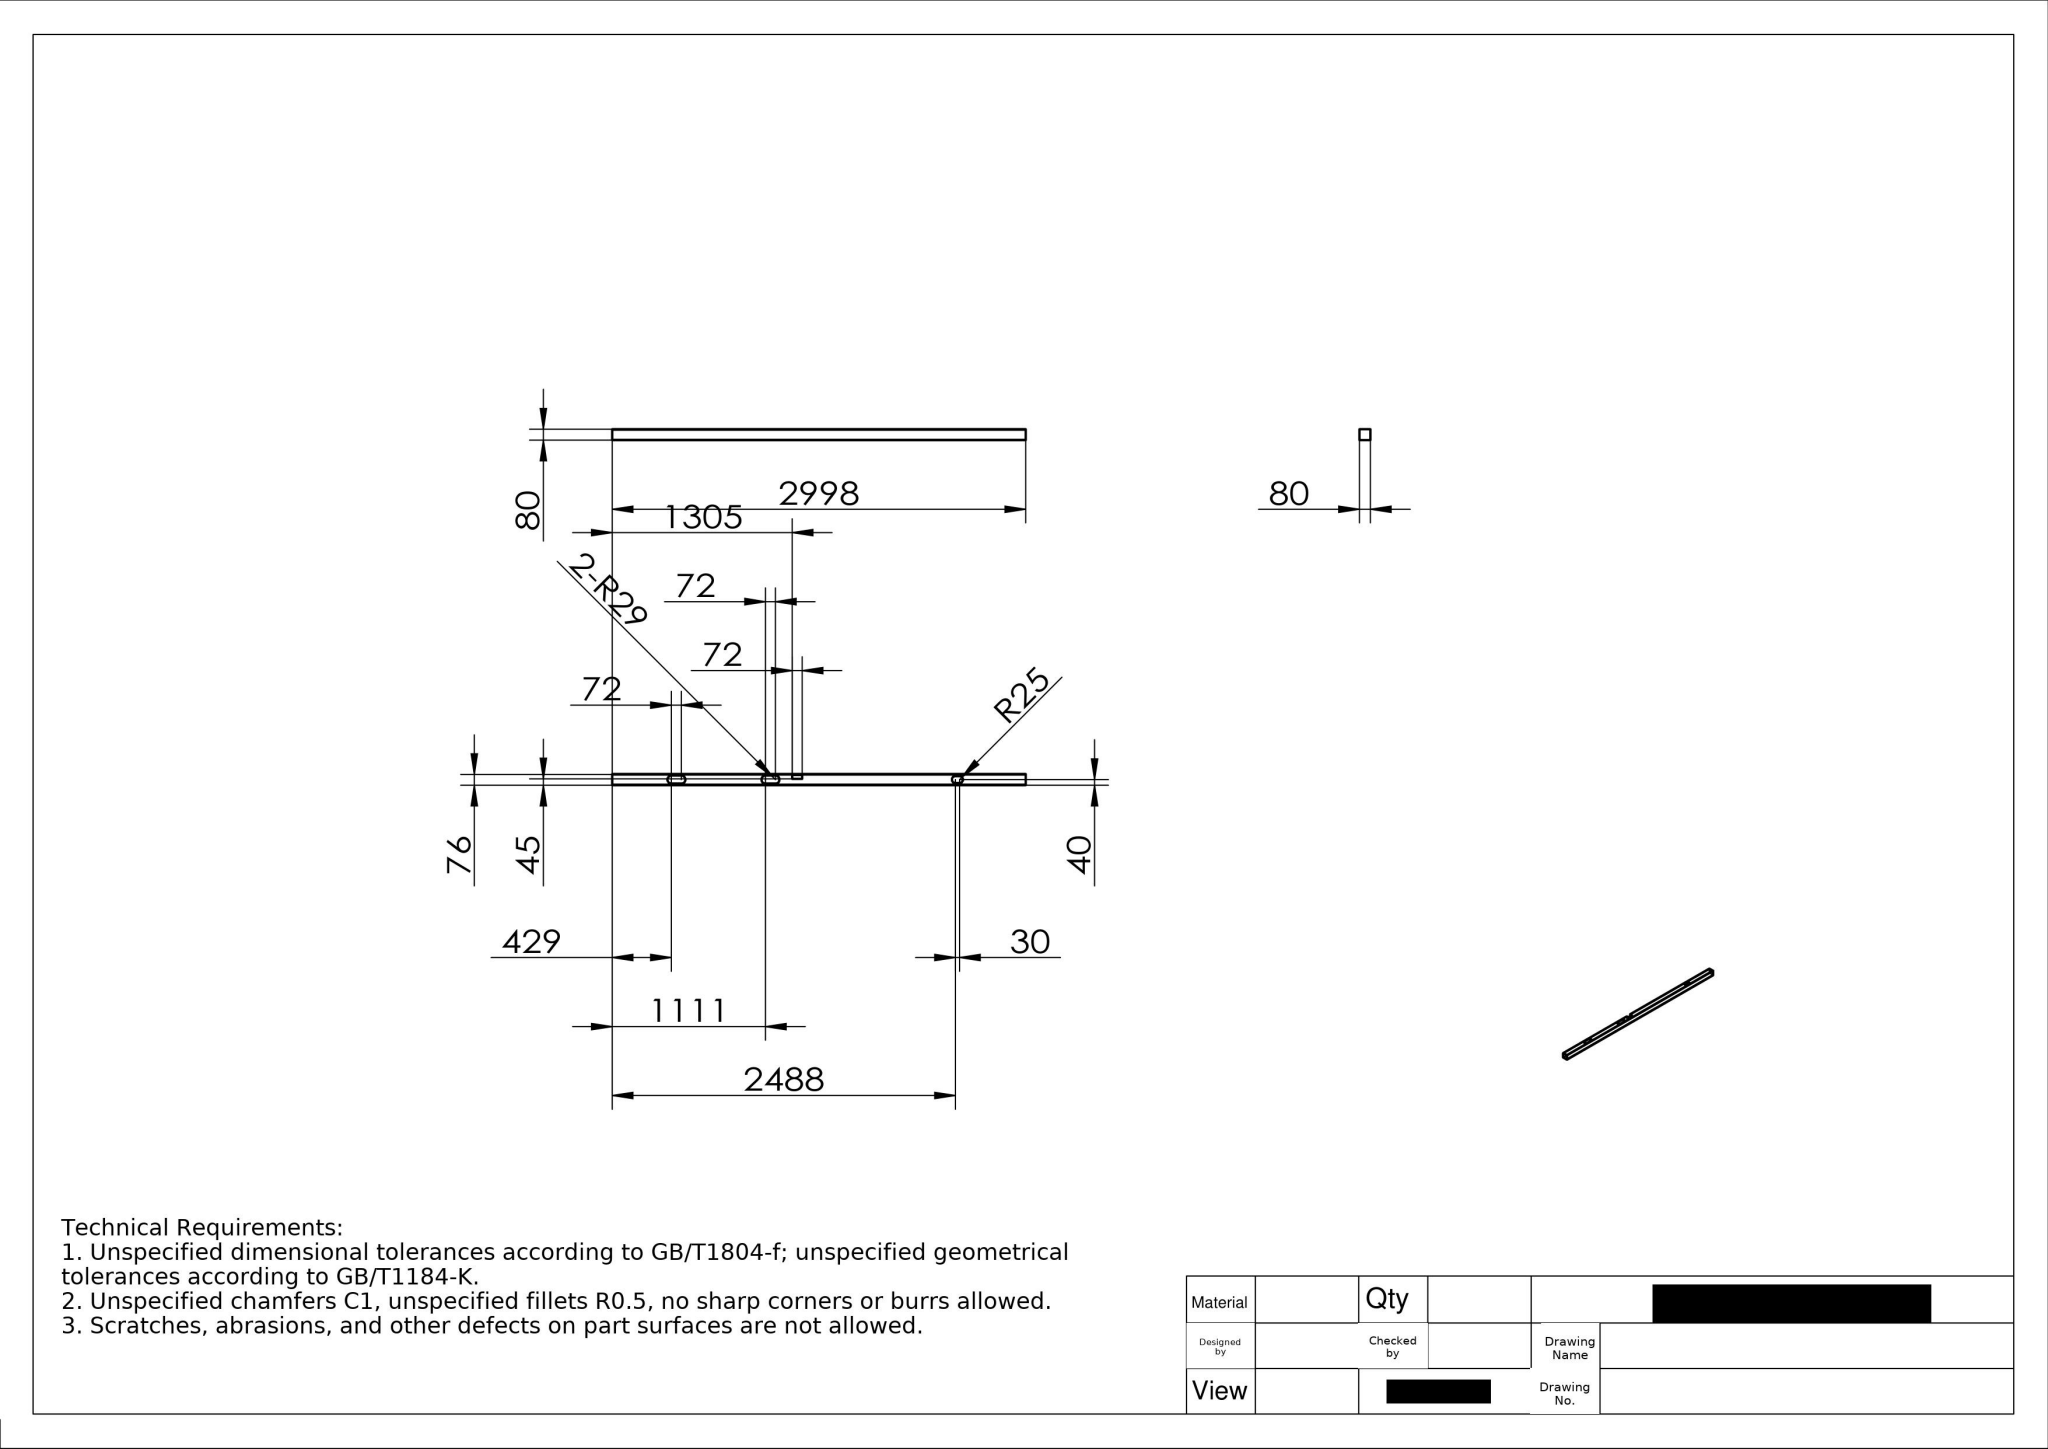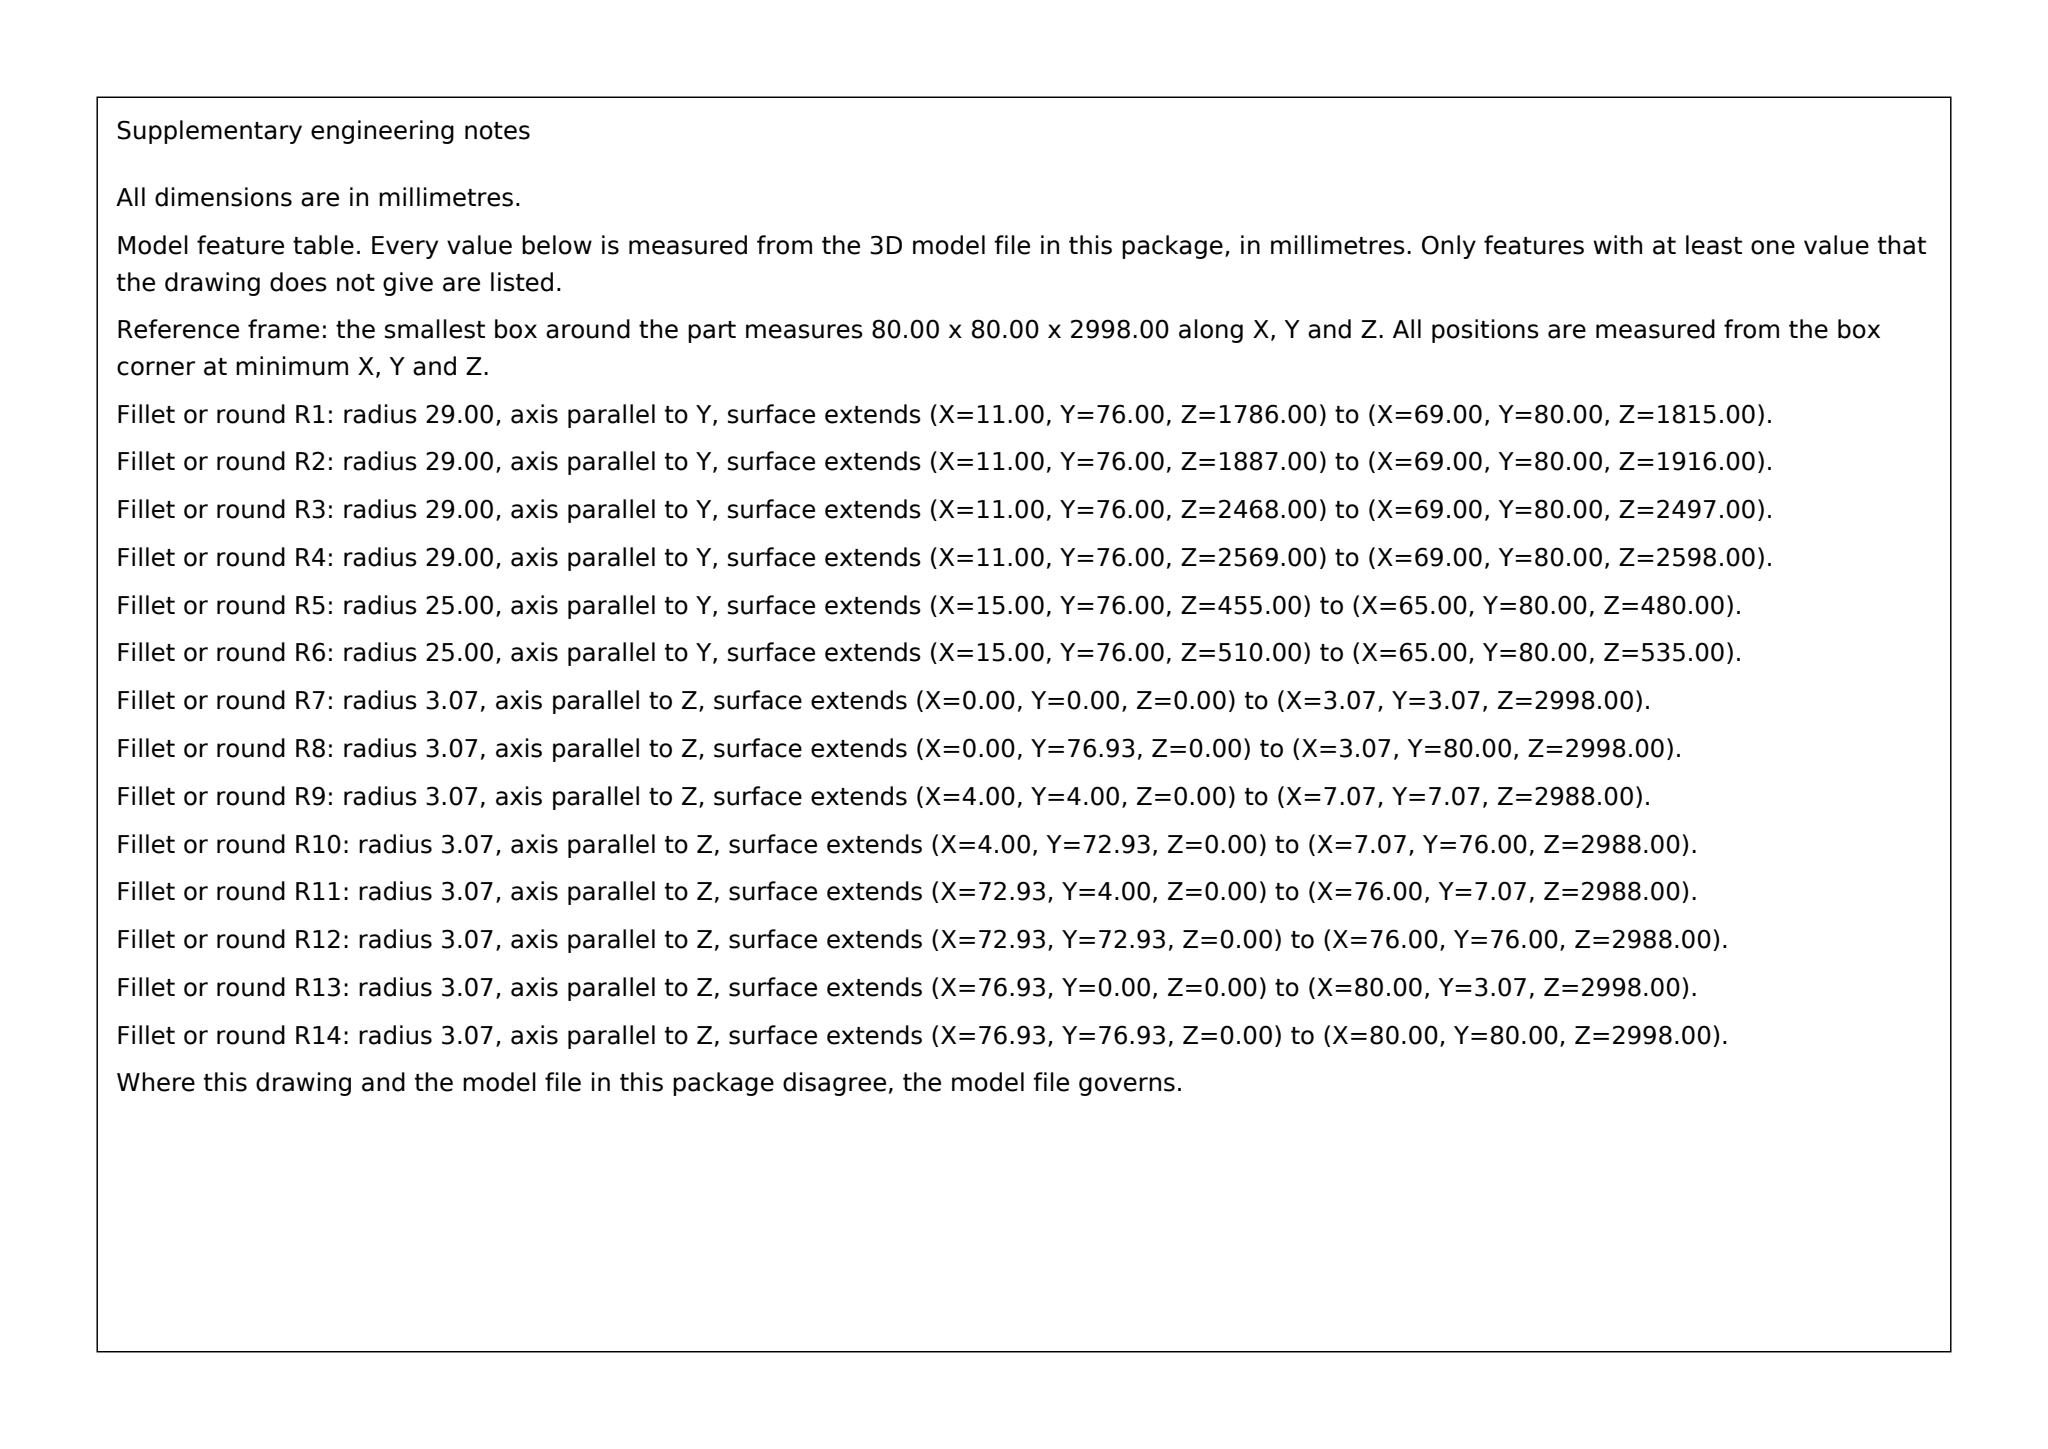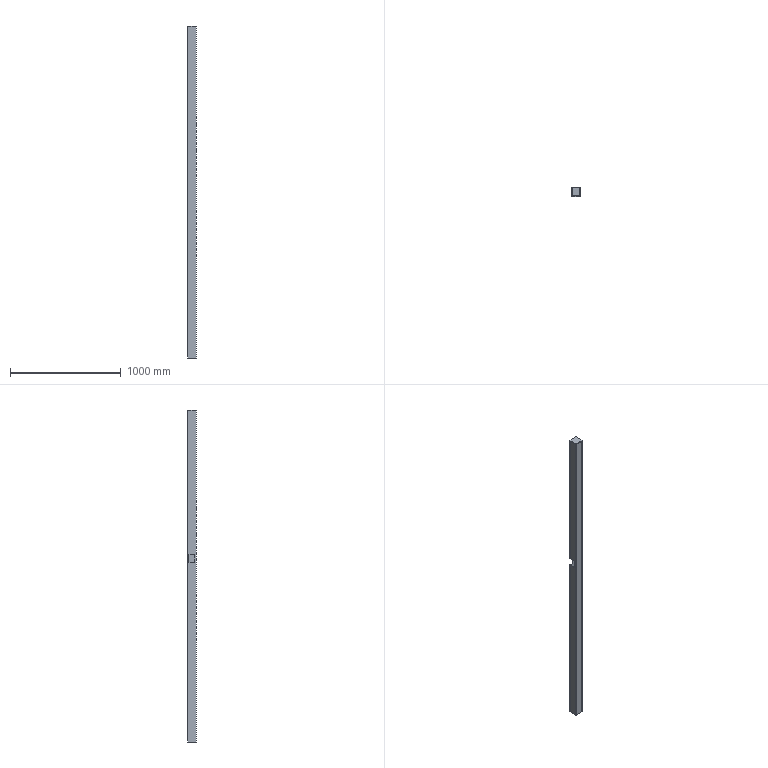Part | SolidWorks | mm | 1 solid | 40 faces | box 80 x 80 x 2998 mm | volume 3602720 mm3 | plane 21 | cylinder 19 | commonest cylinder face diameters 6.148 x10 58 x6 50 x3
build123d program:
from build123d import *

# Parameters (mm, degrees)
BASE_EXTRUDE_DEPTH  = 2998
SKETCH8_W           = 78.199
SKETCH8_H           = 78.199
BOSS_EXTRUDE3_DEPTH = 10
CUT_EXTRUDE6_DEPTH  = 10
SKETCH12_W          = 50
SKETCH12_H          = 72
CUT_EXTRUDE7_DEPTH  = 60
CUT_EXTRUDE8_DEPTH  = 10


with BuildPart() as part:
    # Sketch1 → Base-Extrude (new body)
    with BuildSketch(Plane.XY):
        with BuildLine():
            Line((-36.926, 40), (36.926, 40))
            ThreePointArc((36.926, 40), (39.1, 39.1), (40, 36.926))
            Line((40, 36.926), (40, -36.926))
            ThreePointArc((40, -36.926), (39.1, -39.1), (36.926, -40))
            Line((36.926, -40), (-36.926, -40))
            ThreePointArc((-36.926, -40), (-39.1, -39.1), (-40, -36.926))
            Line((-40, -36.926), (-40, 36.926))
            ThreePointArc((-40, 36.926), (-39.1, 39.1), (-36.926, 40))
        make_face()
        with BuildLine():
            Line((-32.926, 36), (32.926, 36))
            ThreePointArc((32.926, 36), (35.1, 35.1), (36, 32.926))
            Line((36, 32.926), (36, -32.926))
            ThreePointArc((36, -32.926), (35.1, -35.1), (32.926, -36))
            Line((32.926, -36), (-32.926, -36))
            ThreePointArc((-32.926, -36), (-35.1, -35.1), (-36, -32.926))
            Line((-36, -32.926), (-36, 32.926))
            ThreePointArc((-36, 32.926), (-35.1, 35.1), (-32.926, 36))
        make_face(mode=Mode.SUBTRACT)
    extrude(amount=BASE_EXTRUDE_DEPTH)

    # Sketch8 → Boss-Extrude3 (add)
    with BuildSketch(Plane.XY.offset(2998)):
        Rectangle(SKETCH8_W, SKETCH8_H)
    extrude(amount=-BOSS_EXTRUDE3_DEPTH)

    # Sketch11 → Cut-Extrude6 (cut)
    with BuildSketch(Plane(origin=(0, 40, 0), x_dir=(1, 0, 0), z_dir=(0, 1, 0))):
        with BuildLine():
            Line((-29, -2569), (-29, -2497))
            ThreePointArc((-29, -2497), (0, -2468), (29, -2497))
            Line((29, -2497), (29, -2569))
            ThreePointArc((29, -2569), (0, -2598), (-29, -2569))
        make_face()
        with BuildLine():
            Line((-29, -1887), (-29, -1815))
            ThreePointArc((-29, -1815), (0, -1786), (29, -1815))
            Line((29, -1815), (29, -1887))
            ThreePointArc((29, -1887), (0, -1916), (-29, -1887))
        make_face()
    extrude(amount=-CUT_EXTRUDE6_DEPTH, mode=Mode.SUBTRACT)

    # Sketch12 → Cut-Extrude7 (cut)
    with BuildSketch(Plane(origin=(0, 40, 0), x_dir=(1, 0, 0), z_dir=(0, 1, 0))):
        with Locations((-30, -1657)):
            Rectangle(SKETCH12_W, SKETCH12_H)
    extrude(amount=-CUT_EXTRUDE7_DEPTH, mode=Mode.SUBTRACT)

    # Sketch13 → Cut-Extrude8 (cut)
    with BuildSketch(Plane(origin=(0, 40, 0), x_dir=(1, 0, 0), z_dir=(0, 1, 0))):
        with BuildLine():
            Line((-25, -510), (-25, -480))
            ThreePointArc((-25, -480), (0, -455), (25, -480))
            Line((25, -480), (25, -510))
            ThreePointArc((25, -510), (0, -535), (-25, -510))
        make_face()
    extrude(amount=-CUT_EXTRUDE8_DEPTH, mode=Mode.SUBTRACT)


solid = part.part